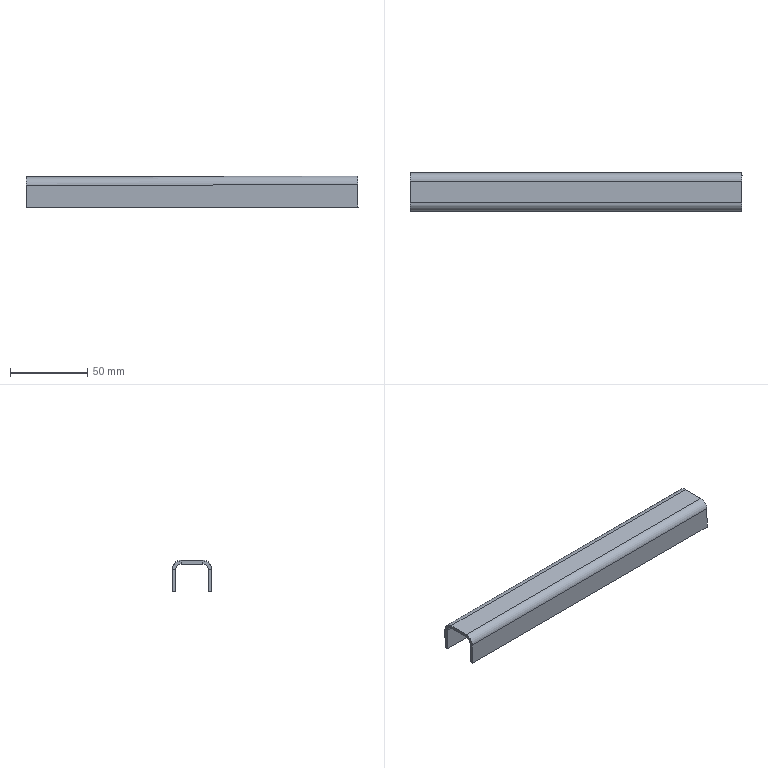Component | SolidWorks | LeftRearDoor-1_RearDoorUpperAndLowerReinforcementBar-1 | 1 solid | 22 faces | box 215.05 x 25 x 20.54 mm | volume 24569 mm3 | plane 18 | cylinder 4 | commonest cylinder face diameters 11 x2 7 x2 | material Malleable Cast Iron
STEP:
#1=COLOUR_RGB('',0.7922,0.8196,0.9333);
#2=FILL_AREA_STYLE_COLOUR('',#1);
#3=FILL_AREA_STYLE('',(#2));
#4=SURFACE_STYLE_FILL_AREA(#3);
#5=SURFACE_SIDE_STYLE('',(#4));
#6=SURFACE_STYLE_USAGE(.BOTH.,#5);
#7=PRESENTATION_STYLE_ASSIGNMENT((#6));
#8=CARTESIAN_POINT('',(9.361,73.502,-6.524));
#9=VERTEX_POINT('',#8);
#10=CARTESIAN_POINT('',(9.361,73.502,-6.603));
#11=VERTEX_POINT('',#10);
#12=CARTESIAN_POINT('',(9.361,73.502,-6.524));
#13=DIRECTION('',(0.002502,0.,-1.));
#14=VECTOR('',#13,39.37);
#15=LINE('',#12,#14);
#16=EDGE_CURVE('',#9,#11,#15,.T.);
#17=ORIENTED_EDGE('',*,*,#16,.F.);
#18=CARTESIAN_POINT('',(9.362,73.286,-6.741));
#19=VERTEX_POINT('',#18);
#20=CARTESIAN_POINT('',(9.362,73.502,-6.741));
#21=DIRECTION('',(-1.,-0.,-0.002502));
#22=DIRECTION('',(0.002502,0.,-1.));
#23=AXIS2_PLACEMENT_3D('',#20,#21,#22);
#24=CIRCLE('',#23,0.2165);
#25=EDGE_CURVE('',#19,#9,#24,.T.);
#26=ORIENTED_EDGE('',*,*,#25,.F.);
#27=CARTESIAN_POINT('',(9.362,73.365,-6.741));
#28=VERTEX_POINT('',#27);
#29=CARTESIAN_POINT('',(9.362,73.365,-6.741));
#30=DIRECTION('',(0.,-1.,-0.));
#31=VECTOR('',#30,39.37);
#32=LINE('',#29,#31);
#33=EDGE_CURVE('',#28,#19,#32,.T.);
#34=ORIENTED_EDGE('',*,*,#33,.F.);
#35=CARTESIAN_POINT('',(9.362,73.502,-6.741));
#36=DIRECTION('',(-1.,-0.,-0.002502));
#37=DIRECTION('',(0.,1.,0.));
#38=AXIS2_PLACEMENT_3D('',#35,#36,#37);
#39=CIRCLE('',#38,0.1378);
#40=EDGE_CURVE('',#28,#11,#39,.T.);
#41=ORIENTED_EDGE('',*,*,#40,.T.);
#42=EDGE_LOOP('',(#17,#26,#34,#41));
#43=FACE_OUTER_BOUND('',#42,.T.);
#44=CARTESIAN_POINT('',(9.361,73.502,-6.524));
#45=DIRECTION('',(1.,0.,0.002502));
#46=DIRECTION('',(0.002502,0.,-1.));
#47=AXIS2_PLACEMENT_3D('',#44,#45,#46);
#48=PLANE('',#47);
#49=ADVANCED_FACE('',(#43),#48,.T.);
#50=CARTESIAN_POINT('',(9.361,74.054,-6.524));
#51=VERTEX_POINT('',#50);
#52=CARTESIAN_POINT('',(9.361,73.286,-6.524));
#53=DIRECTION('',(-0.,1.,0.));
#54=VECTOR('',#53,39.37);
#55=LINE('',#52,#54);
#56=EDGE_CURVE('',#9,#51,#55,.T.);
#57=ORIENTED_EDGE('',*,*,#56,.F.);
#58=ORIENTED_EDGE('',*,*,#16,.T.);
#59=CARTESIAN_POINT('',(9.361,74.054,-6.603));
#60=VERTEX_POINT('',#59);
#61=CARTESIAN_POINT('',(9.361,73.286,-6.603));
#62=DIRECTION('',(-0.,1.,0.));
#63=VECTOR('',#62,39.37);
#64=LINE('',#61,#63);
#65=EDGE_CURVE('',#11,#60,#64,.T.);
#66=ORIENTED_EDGE('',*,*,#65,.T.);
#67=CARTESIAN_POINT('',(9.361,74.054,-6.603));
#68=DIRECTION('',(-0.002502,-0.,1.));
#69=VECTOR('',#68,39.37);
#70=LINE('',#67,#69);
#71=EDGE_CURVE('',#60,#51,#70,.T.);
#72=ORIENTED_EDGE('',*,*,#71,.T.);
#73=EDGE_LOOP('',(#57,#58,#66,#72));
#74=FACE_OUTER_BOUND('',#73,.T.);
#75=CARTESIAN_POINT('',(9.362,73.365,-6.741));
#76=DIRECTION('',(1.,0.,0.002502));
#77=DIRECTION('',(0.002502,0.,-1.));
#78=AXIS2_PLACEMENT_3D('',#75,#76,#77);
#79=PLANE('',#78);
#80=ADVANCED_FACE('',(#74),#79,.T.);
#81=CARTESIAN_POINT('',(0.897,73.286,-6.762));
#82=VERTEX_POINT('',#81);
#83=CARTESIAN_POINT('',(0.897,73.365,-6.762));
#84=VERTEX_POINT('',#83);
#85=CARTESIAN_POINT('',(0.897,73.286,-6.762));
#86=DIRECTION('',(-0.,1.,0.));
#87=VECTOR('',#86,39.37);
#88=LINE('',#85,#87);
#89=EDGE_CURVE('',#82,#84,#88,.T.);
#90=ORIENTED_EDGE('',*,*,#89,.F.);
#91=CARTESIAN_POINT('',(0.8965,73.502,-6.545));
#92=VERTEX_POINT('',#91);
#93=CARTESIAN_POINT('',(0.897,73.502,-6.762));
#94=DIRECTION('',(-1.,-0.,-0.002502));
#95=DIRECTION('',(0.002502,0.,-1.));
#96=AXIS2_PLACEMENT_3D('',#93,#94,#95);
#97=CIRCLE('',#96,0.2165);
#98=EDGE_CURVE('',#82,#92,#97,.T.);
#99=ORIENTED_EDGE('',*,*,#98,.T.);
#100=CARTESIAN_POINT('',(0.8967,73.502,-6.624));
#101=VERTEX_POINT('',#100);
#102=CARTESIAN_POINT('',(0.8967,73.502,-6.624));
#103=DIRECTION('',(-0.002502,-0.,1.));
#104=VECTOR('',#103,39.37);
#105=LINE('',#102,#104);
#106=EDGE_CURVE('',#101,#92,#105,.T.);
#107=ORIENTED_EDGE('',*,*,#106,.F.);
#108=CARTESIAN_POINT('',(0.897,73.502,-6.762));
#109=DIRECTION('',(-1.,-0.,-0.002502));
#110=DIRECTION('',(-0.,1.,0.));
#111=AXIS2_PLACEMENT_3D('',#108,#109,#110);
#112=CIRCLE('',#111,0.1378);
#113=EDGE_CURVE('',#84,#101,#112,.T.);
#114=ORIENTED_EDGE('',*,*,#113,.F.);
#115=EDGE_LOOP('',(#90,#99,#107,#114));
#116=FACE_OUTER_BOUND('',#115,.T.);
#117=CARTESIAN_POINT('',(0.897,73.286,-6.762));
#118=DIRECTION('',(-1.,-0.,-0.002502));
#119=DIRECTION('',(-0.002502,-0.,1.));
#120=AXIS2_PLACEMENT_3D('',#117,#118,#119);
#121=PLANE('',#120);
#122=ADVANCED_FACE('',(#116),#121,.T.);
#123=CARTESIAN_POINT('',(0.8984,73.286,-7.333));
#124=VERTEX_POINT('',#123);
#125=CARTESIAN_POINT('',(0.8984,73.286,-7.333));
#126=DIRECTION('',(-0.002502,-0.,1.));
#127=VECTOR('',#126,39.37);
#128=LINE('',#125,#127);
#129=EDGE_CURVE('',#124,#82,#128,.T.);
#130=ORIENTED_EDGE('',*,*,#129,.T.);
#131=ORIENTED_EDGE('',*,*,#89,.T.);
#132=CARTESIAN_POINT('',(0.8984,73.365,-7.333));
#133=VERTEX_POINT('',#132);
#134=CARTESIAN_POINT('',(0.8984,73.365,-7.333));
#135=DIRECTION('',(-0.002502,-0.,1.));
#136=VECTOR('',#135,39.37);
#137=LINE('',#134,#136);
#138=EDGE_CURVE('',#133,#84,#137,.T.);
#139=ORIENTED_EDGE('',*,*,#138,.F.);
#140=CARTESIAN_POINT('',(0.8984,73.365,-7.333));
#141=DIRECTION('',(0.,-1.,-0.));
#142=VECTOR('',#141,39.37);
#143=LINE('',#140,#142);
#144=EDGE_CURVE('',#133,#124,#143,.T.);
#145=ORIENTED_EDGE('',*,*,#144,.T.);
#146=EDGE_LOOP('',(#130,#131,#139,#145));
#147=FACE_OUTER_BOUND('',#146,.T.);
#148=CARTESIAN_POINT('',(0.8967,73.502,-6.624));
#149=DIRECTION('',(-1.,-0.,-0.002502));
#150=DIRECTION('',(-0.002502,-0.,1.));
#151=AXIS2_PLACEMENT_3D('',#148,#149,#150);
#152=PLANE('',#151);
#153=ADVANCED_FACE('',(#147),#152,.T.);
#154=CARTESIAN_POINT('',(9.362,74.27,-6.741));
#155=VERTEX_POINT('',#154);
#156=CARTESIAN_POINT('',(9.362,74.191,-6.741));
#157=VERTEX_POINT('',#156);
#158=CARTESIAN_POINT('',(9.362,74.27,-6.741));
#159=DIRECTION('',(0.,-1.,-0.));
#160=VECTOR('',#159,39.37);
#161=LINE('',#158,#160);
#162=EDGE_CURVE('',#155,#157,#161,.T.);
#163=ORIENTED_EDGE('',*,*,#162,.F.);
#164=CARTESIAN_POINT('',(9.362,74.054,-6.741));
#165=DIRECTION('',(-1.,-0.,-0.002502));
#166=DIRECTION('',(0.002502,0.,-1.));
#167=AXIS2_PLACEMENT_3D('',#164,#165,#166);
#168=CIRCLE('',#167,0.2165);
#169=EDGE_CURVE('',#51,#155,#168,.T.);
#170=ORIENTED_EDGE('',*,*,#169,.F.);
#171=ORIENTED_EDGE('',*,*,#71,.F.);
#172=CARTESIAN_POINT('',(9.362,74.054,-6.741));
#173=DIRECTION('',(-1.,-0.,-0.002502));
#174=DIRECTION('',(0.,1.,0.));
#175=AXIS2_PLACEMENT_3D('',#172,#173,#174);
#176=CIRCLE('',#175,0.1378);
#177=EDGE_CURVE('',#60,#157,#176,.T.);
#178=ORIENTED_EDGE('',*,*,#177,.T.);
#179=EDGE_LOOP('',(#163,#170,#171,#178));
#180=FACE_OUTER_BOUND('',#179,.T.);
#181=CARTESIAN_POINT('',(9.362,74.27,-6.741));
#182=DIRECTION('',(1.,0.,0.002502));
#183=DIRECTION('',(0.002502,0.,-1.));
#184=AXIS2_PLACEMENT_3D('',#181,#182,#183);
#185=PLANE('',#184);
#186=ADVANCED_FACE('',(#180),#185,.T.);
#187=CARTESIAN_POINT('',(9.363,74.27,-7.312));
#188=VERTEX_POINT('',#187);
#189=CARTESIAN_POINT('',(9.361,74.27,-6.524));
#190=DIRECTION('',(0.002502,0.,-1.));
#191=VECTOR('',#190,39.37);
#192=LINE('',#189,#191);
#193=EDGE_CURVE('',#155,#188,#192,.T.);
#194=ORIENTED_EDGE('',*,*,#193,.F.);
#195=ORIENTED_EDGE('',*,*,#162,.T.);
#196=CARTESIAN_POINT('',(9.363,74.191,-7.312));
#197=VERTEX_POINT('',#196);
#198=CARTESIAN_POINT('',(9.361,74.191,-6.524));
#199=DIRECTION('',(0.002502,0.,-1.));
#200=VECTOR('',#199,39.37);
#201=LINE('',#198,#200);
#202=EDGE_CURVE('',#157,#197,#201,.T.);
#203=ORIENTED_EDGE('',*,*,#202,.T.);
#204=CARTESIAN_POINT('',(9.363,74.27,-7.312));
#205=DIRECTION('',(0.,-1.,-0.));
#206=VECTOR('',#205,39.37);
#207=LINE('',#204,#206);
#208=EDGE_CURVE('',#188,#197,#207,.T.);
#209=ORIENTED_EDGE('',*,*,#208,.F.);
#210=EDGE_LOOP('',(#194,#195,#203,#209));
#211=FACE_OUTER_BOUND('',#210,.T.);
#212=CARTESIAN_POINT('',(9.361,74.054,-6.603));
#213=DIRECTION('',(1.,0.,0.002502));
#214=DIRECTION('',(0.002502,0.,-1.));
#215=AXIS2_PLACEMENT_3D('',#212,#213,#214);
#216=PLANE('',#215);
#217=ADVANCED_FACE('',(#211),#216,.T.);
#218=CARTESIAN_POINT('',(0.8965,74.054,-6.545));
#219=VERTEX_POINT('',#218);
#220=CARTESIAN_POINT('',(0.8967,74.054,-6.624));
#221=VERTEX_POINT('',#220);
#222=CARTESIAN_POINT('',(0.8965,74.054,-6.545));
#223=DIRECTION('',(0.002502,0.,-1.));
#224=VECTOR('',#223,39.37);
#225=LINE('',#222,#224);
#226=EDGE_CURVE('',#219,#221,#225,.T.);
#227=ORIENTED_EDGE('',*,*,#226,.F.);
#228=CARTESIAN_POINT('',(0.897,74.27,-6.762));
#229=VERTEX_POINT('',#228);
#230=CARTESIAN_POINT('',(0.897,74.054,-6.762));
#231=DIRECTION('',(-1.,-0.,-0.002502));
#232=DIRECTION('',(0.002502,0.,-1.));
#233=AXIS2_PLACEMENT_3D('',#230,#231,#232);
#234=CIRCLE('',#233,0.2165);
#235=EDGE_CURVE('',#219,#229,#234,.T.);
#236=ORIENTED_EDGE('',*,*,#235,.T.);
#237=CARTESIAN_POINT('',(0.897,74.191,-6.762));
#238=VERTEX_POINT('',#237);
#239=CARTESIAN_POINT('',(0.897,74.191,-6.762));
#240=DIRECTION('',(-0.,1.,0.));
#241=VECTOR('',#240,39.37);
#242=LINE('',#239,#241);
#243=EDGE_CURVE('',#238,#229,#242,.T.);
#244=ORIENTED_EDGE('',*,*,#243,.F.);
#245=CARTESIAN_POINT('',(0.897,74.054,-6.762));
#246=DIRECTION('',(-1.,-0.,-0.002502));
#247=DIRECTION('',(-0.,1.,0.));
#248=AXIS2_PLACEMENT_3D('',#245,#246,#247);
#249=CIRCLE('',#248,0.1378);
#250=EDGE_CURVE('',#221,#238,#249,.T.);
#251=ORIENTED_EDGE('',*,*,#250,.F.);
#252=EDGE_LOOP('',(#227,#236,#244,#251));
#253=FACE_OUTER_BOUND('',#252,.T.);
#254=CARTESIAN_POINT('',(0.8965,74.054,-6.545));
#255=DIRECTION('',(-1.,-0.,-0.002502));
#256=DIRECTION('',(-0.002502,-0.,1.));
#257=AXIS2_PLACEMENT_3D('',#254,#255,#256);
#258=PLANE('',#257);
#259=ADVANCED_FACE('',(#253),#258,.T.);
#260=CARTESIAN_POINT('',(0.8965,73.286,-6.545));
#261=DIRECTION('',(-0.,1.,0.));
#262=VECTOR('',#261,39.37);
#263=LINE('',#260,#262);
#264=EDGE_CURVE('',#92,#219,#263,.T.);
#265=ORIENTED_EDGE('',*,*,#264,.T.);
#266=ORIENTED_EDGE('',*,*,#226,.T.);
#267=CARTESIAN_POINT('',(0.8967,73.286,-6.624));
#268=DIRECTION('',(-0.,1.,0.));
#269=VECTOR('',#268,39.37);
#270=LINE('',#267,#269);
#271=EDGE_CURVE('',#101,#221,#270,.T.);
#272=ORIENTED_EDGE('',*,*,#271,.F.);
#273=ORIENTED_EDGE('',*,*,#106,.T.);
#274=EDGE_LOOP('',(#265,#266,#272,#273));
#275=FACE_OUTER_BOUND('',#274,.T.);
#276=CARTESIAN_POINT('',(0.897,74.191,-6.762));
#277=DIRECTION('',(-1.,-0.,-0.002502));
#278=DIRECTION('',(-0.002502,-0.,1.));
#279=AXIS2_PLACEMENT_3D('',#276,#277,#278);
#280=PLANE('',#279);
#281=ADVANCED_FACE('',(#275),#280,.T.);
#282=CARTESIAN_POINT('',(0.8984,74.191,-7.333));
#283=VERTEX_POINT('',#282);
#284=CARTESIAN_POINT('',(0.8965,74.191,-6.545));
#285=DIRECTION('',(0.002502,0.,-1.));
#286=VECTOR('',#285,39.37);
#287=LINE('',#284,#286);
#288=EDGE_CURVE('',#238,#283,#287,.T.);
#289=ORIENTED_EDGE('',*,*,#288,.T.);
#290=CARTESIAN_POINT('',(9.363,74.191,-7.312));
#291=DIRECTION('',(-1.,-0.,-0.002502));
#292=VECTOR('',#291,39.37);
#293=LINE('',#290,#292);
#294=EDGE_CURVE('',#197,#283,#293,.T.);
#295=ORIENTED_EDGE('',*,*,#294,.F.);
#296=ORIENTED_EDGE('',*,*,#202,.F.);
#297=CARTESIAN_POINT('',(9.362,74.191,-6.741));
#298=DIRECTION('',(-1.,-0.,-0.002502));
#299=VECTOR('',#298,39.37);
#300=LINE('',#297,#299);
#301=EDGE_CURVE('',#157,#238,#300,.T.);
#302=ORIENTED_EDGE('',*,*,#301,.T.);
#303=EDGE_LOOP('',(#289,#295,#296,#302));
#304=FACE_OUTER_BOUND('',#303,.T.);
#305=CARTESIAN_POINT('',(9.361,74.191,-6.524));
#306=DIRECTION('',(-0.,1.,0.));
#307=DIRECTION('',(-0.002502,-0.,1.));
#308=AXIS2_PLACEMENT_3D('',#305,#306,#307);
#309=PLANE('',#308);
#310=ADVANCED_FACE('',(#304),#309,.F.);
#311=CARTESIAN_POINT('',(0.8984,74.27,-7.333));
#312=VERTEX_POINT('',#311);
#313=CARTESIAN_POINT('',(0.8984,74.27,-7.333));
#314=DIRECTION('',(0.,-1.,-0.));
#315=VECTOR('',#314,39.37);
#316=LINE('',#313,#315);
#317=EDGE_CURVE('',#312,#283,#316,.T.);
#318=ORIENTED_EDGE('',*,*,#317,.F.);
#319=CARTESIAN_POINT('',(9.363,74.27,-7.312));
#320=DIRECTION('',(-1.,-0.,-0.002502));
#321=VECTOR('',#320,39.37);
#322=LINE('',#319,#321);
#323=EDGE_CURVE('',#188,#312,#322,.T.);
#324=ORIENTED_EDGE('',*,*,#323,.F.);
#325=ORIENTED_EDGE('',*,*,#208,.T.);
#326=ORIENTED_EDGE('',*,*,#294,.T.);
#327=EDGE_LOOP('',(#318,#324,#325,#326));
#328=FACE_OUTER_BOUND('',#327,.T.);
#329=CARTESIAN_POINT('',(9.363,74.27,-7.312));
#330=DIRECTION('',(0.002502,0.,-1.));
#331=DIRECTION('',(-0.,1.,0.));
#332=AXIS2_PLACEMENT_3D('',#329,#330,#331);
#333=PLANE('',#332);
#334=ADVANCED_FACE('',(#328),#333,.T.);
#335=CARTESIAN_POINT('',(0.8965,74.27,-6.545));
#336=DIRECTION('',(0.002502,0.,-1.));
#337=VECTOR('',#336,39.37);
#338=LINE('',#335,#337);
#339=EDGE_CURVE('',#229,#312,#338,.T.);
#340=ORIENTED_EDGE('',*,*,#339,.F.);
#341=CARTESIAN_POINT('',(9.362,74.27,-6.741));
#342=DIRECTION('',(-1.,-0.,-0.002502));
#343=VECTOR('',#342,39.37);
#344=LINE('',#341,#343);
#345=EDGE_CURVE('',#155,#229,#344,.T.);
#346=ORIENTED_EDGE('',*,*,#345,.F.);
#347=ORIENTED_EDGE('',*,*,#193,.T.);
#348=ORIENTED_EDGE('',*,*,#323,.T.);
#349=EDGE_LOOP('',(#340,#346,#347,#348));
#350=FACE_OUTER_BOUND('',#349,.T.);
#351=CARTESIAN_POINT('',(9.361,74.27,-6.524));
#352=DIRECTION('',(-0.,1.,0.));
#353=DIRECTION('',(-0.002502,-0.,1.));
#354=AXIS2_PLACEMENT_3D('',#351,#352,#353);
#355=PLANE('',#354);
#356=ADVANCED_FACE('',(#350),#355,.T.);
#357=ORIENTED_EDGE('',*,*,#235,.F.);
#358=CARTESIAN_POINT('',(9.361,74.054,-6.524));
#359=DIRECTION('',(-1.,-0.,-0.002502));
#360=VECTOR('',#359,39.37);
#361=LINE('',#358,#360);
#362=EDGE_CURVE('',#51,#219,#361,.T.);
#363=ORIENTED_EDGE('',*,*,#362,.F.);
#364=ORIENTED_EDGE('',*,*,#169,.T.);
#365=ORIENTED_EDGE('',*,*,#345,.T.);
#366=EDGE_LOOP('',(#357,#363,#364,#365));
#367=FACE_OUTER_BOUND('',#366,.T.);
#368=CARTESIAN_POINT('',(9.362,74.054,-6.741));
#369=DIRECTION('',(-1.,-0.,-0.002502));
#370=DIRECTION('',(-0.002502,0.,1.));
#371=AXIS2_PLACEMENT_3D('',#368,#369,#370);
#372=CYLINDRICAL_SURFACE('',#371,0.2165);
#373=ADVANCED_FACE('',(#367),#372,.T.);
#374=ORIENTED_EDGE('',*,*,#264,.F.);
#375=CARTESIAN_POINT('',(9.361,73.502,-6.524));
#376=DIRECTION('',(-1.,-0.,-0.002502));
#377=VECTOR('',#376,39.37);
#378=LINE('',#375,#377);
#379=EDGE_CURVE('',#9,#92,#378,.T.);
#380=ORIENTED_EDGE('',*,*,#379,.F.);
#381=ORIENTED_EDGE('',*,*,#56,.T.);
#382=ORIENTED_EDGE('',*,*,#362,.T.);
#383=EDGE_LOOP('',(#374,#380,#381,#382));
#384=FACE_OUTER_BOUND('',#383,.T.);
#385=CARTESIAN_POINT('',(9.361,73.286,-6.524));
#386=DIRECTION('',(-0.002502,-0.,1.));
#387=DIRECTION('',(0.,-1.,-0.));
#388=AXIS2_PLACEMENT_3D('',#385,#386,#387);
#389=PLANE('',#388);
#390=ADVANCED_FACE('',(#384),#389,.T.);
#391=ORIENTED_EDGE('',*,*,#98,.F.);
#392=CARTESIAN_POINT('',(9.362,73.286,-6.741));
#393=DIRECTION('',(-1.,-0.,-0.002502));
#394=VECTOR('',#393,39.37);
#395=LINE('',#392,#394);
#396=EDGE_CURVE('',#19,#82,#395,.T.);
#397=ORIENTED_EDGE('',*,*,#396,.F.);
#398=ORIENTED_EDGE('',*,*,#25,.T.);
#399=ORIENTED_EDGE('',*,*,#379,.T.);
#400=EDGE_LOOP('',(#391,#397,#398,#399));
#401=FACE_OUTER_BOUND('',#400,.T.);
#402=CARTESIAN_POINT('',(9.362,73.502,-6.741));
#403=DIRECTION('',(-1.,-0.,-0.002502));
#404=DIRECTION('',(-0.002502,0.,1.));
#405=AXIS2_PLACEMENT_3D('',#402,#403,#404);
#406=CYLINDRICAL_SURFACE('',#405,0.2165);
#407=ADVANCED_FACE('',(#401),#406,.T.);
#408=ORIENTED_EDGE('',*,*,#129,.F.);
#409=CARTESIAN_POINT('',(9.363,73.286,-7.312));
#410=VERTEX_POINT('',#409);
#411=CARTESIAN_POINT('',(9.363,73.286,-7.312));
#412=DIRECTION('',(-1.,-0.,-0.002502));
#413=VECTOR('',#412,39.37);
#414=LINE('',#411,#413);
#415=EDGE_CURVE('',#410,#124,#414,.T.);
#416=ORIENTED_EDGE('',*,*,#415,.F.);
#417=CARTESIAN_POINT('',(9.363,73.286,-7.312));
#418=DIRECTION('',(-0.002502,-0.,1.));
#419=VECTOR('',#418,39.37);
#420=LINE('',#417,#419);
#421=EDGE_CURVE('',#410,#19,#420,.T.);
#422=ORIENTED_EDGE('',*,*,#421,.T.);
#423=ORIENTED_EDGE('',*,*,#396,.T.);
#424=EDGE_LOOP('',(#408,#416,#422,#423));
#425=FACE_OUTER_BOUND('',#424,.T.);
#426=CARTESIAN_POINT('',(9.363,73.286,-7.312));
#427=DIRECTION('',(0.,-1.,-0.));
#428=DIRECTION('',(0.002502,0.,-1.));
#429=AXIS2_PLACEMENT_3D('',#426,#427,#428);
#430=PLANE('',#429);
#431=ADVANCED_FACE('',(#425),#430,.T.);
#432=ORIENTED_EDGE('',*,*,#144,.F.);
#433=CARTESIAN_POINT('',(9.363,73.365,-7.312));
#434=VERTEX_POINT('',#433);
#435=CARTESIAN_POINT('',(9.363,73.365,-7.312));
#436=DIRECTION('',(-1.,-0.,-0.002502));
#437=VECTOR('',#436,39.37);
#438=LINE('',#435,#437);
#439=EDGE_CURVE('',#434,#133,#438,.T.);
#440=ORIENTED_EDGE('',*,*,#439,.F.);
#441=CARTESIAN_POINT('',(9.363,73.365,-7.312));
#442=DIRECTION('',(0.,-1.,-0.));
#443=VECTOR('',#442,39.37);
#444=LINE('',#441,#443);
#445=EDGE_CURVE('',#434,#410,#444,.T.);
#446=ORIENTED_EDGE('',*,*,#445,.T.);
#447=ORIENTED_EDGE('',*,*,#415,.T.);
#448=EDGE_LOOP('',(#432,#440,#446,#447));
#449=FACE_OUTER_BOUND('',#448,.T.);
#450=CARTESIAN_POINT('',(9.363,73.365,-7.312));
#451=DIRECTION('',(0.002502,0.,-1.));
#452=DIRECTION('',(-0.,1.,0.));
#453=AXIS2_PLACEMENT_3D('',#450,#451,#452);
#454=PLANE('',#453);
#455=ADVANCED_FACE('',(#449),#454,.T.);
#456=ORIENTED_EDGE('',*,*,#138,.T.);
#457=CARTESIAN_POINT('',(9.362,73.365,-6.741));
#458=DIRECTION('',(-1.,-0.,-0.002502));
#459=VECTOR('',#458,39.37);
#460=LINE('',#457,#459);
#461=EDGE_CURVE('',#28,#84,#460,.T.);
#462=ORIENTED_EDGE('',*,*,#461,.F.);
#463=CARTESIAN_POINT('',(9.363,73.365,-7.312));
#464=DIRECTION('',(-0.002502,-0.,1.));
#465=VECTOR('',#464,39.37);
#466=LINE('',#463,#465);
#467=EDGE_CURVE('',#434,#28,#466,.T.);
#468=ORIENTED_EDGE('',*,*,#467,.F.);
#469=ORIENTED_EDGE('',*,*,#439,.T.);
#470=EDGE_LOOP('',(#456,#462,#468,#469));
#471=FACE_OUTER_BOUND('',#470,.T.);
#472=CARTESIAN_POINT('',(9.363,73.365,-7.312));
#473=DIRECTION('',(0.,-1.,-0.));
#474=DIRECTION('',(0.002502,0.,-1.));
#475=AXIS2_PLACEMENT_3D('',#472,#473,#474);
#476=PLANE('',#475);
#477=ADVANCED_FACE('',(#471),#476,.F.);
#478=ORIENTED_EDGE('',*,*,#113,.T.);
#479=CARTESIAN_POINT('',(9.361,73.502,-6.603));
#480=DIRECTION('',(-1.,-0.,-0.002502));
#481=VECTOR('',#480,39.37);
#482=LINE('',#479,#481);
#483=EDGE_CURVE('',#11,#101,#482,.T.);
#484=ORIENTED_EDGE('',*,*,#483,.F.);
#485=ORIENTED_EDGE('',*,*,#40,.F.);
#486=ORIENTED_EDGE('',*,*,#461,.T.);
#487=EDGE_LOOP('',(#478,#484,#485,#486));
#488=FACE_OUTER_BOUND('',#487,.T.);
#489=CARTESIAN_POINT('',(9.362,73.502,-6.741));
#490=DIRECTION('',(-1.,-0.,-0.002502));
#491=DIRECTION('',(-0.002502,0.,1.));
#492=AXIS2_PLACEMENT_3D('',#489,#490,#491);
#493=CYLINDRICAL_SURFACE('',#492,0.1378);
#494=ADVANCED_FACE('',(#488),#493,.F.);
#495=ORIENTED_EDGE('',*,*,#271,.T.);
#496=CARTESIAN_POINT('',(9.361,74.054,-6.603));
#497=DIRECTION('',(-1.,-0.,-0.002502));
#498=VECTOR('',#497,39.37);
#499=LINE('',#496,#498);
#500=EDGE_CURVE('',#60,#221,#499,.T.);
#501=ORIENTED_EDGE('',*,*,#500,.F.);
#502=ORIENTED_EDGE('',*,*,#65,.F.);
#503=ORIENTED_EDGE('',*,*,#483,.T.);
#504=EDGE_LOOP('',(#495,#501,#502,#503));
#505=FACE_OUTER_BOUND('',#504,.T.);
#506=CARTESIAN_POINT('',(9.361,73.286,-6.603));
#507=DIRECTION('',(-0.002502,-0.,1.));
#508=DIRECTION('',(0.,-1.,-0.));
#509=AXIS2_PLACEMENT_3D('',#506,#507,#508);
#510=PLANE('',#509);
#511=ADVANCED_FACE('',(#505),#510,.F.);
#512=ORIENTED_EDGE('',*,*,#250,.T.);
#513=ORIENTED_EDGE('',*,*,#301,.F.);
#514=ORIENTED_EDGE('',*,*,#177,.F.);
#515=ORIENTED_EDGE('',*,*,#500,.T.);
#516=EDGE_LOOP('',(#512,#513,#514,#515));
#517=FACE_OUTER_BOUND('',#516,.T.);
#518=CARTESIAN_POINT('',(9.362,74.054,-6.741));
#519=DIRECTION('',(-1.,-0.,-0.002502));
#520=DIRECTION('',(-0.002502,0.,1.));
#521=AXIS2_PLACEMENT_3D('',#518,#519,#520);
#522=CYLINDRICAL_SURFACE('',#521,0.1378);
#523=ADVANCED_FACE('',(#517),#522,.F.);
#524=ORIENTED_EDGE('',*,*,#467,.T.);
#525=ORIENTED_EDGE('',*,*,#33,.T.);
#526=ORIENTED_EDGE('',*,*,#421,.F.);
#527=ORIENTED_EDGE('',*,*,#445,.F.);
#528=EDGE_LOOP('',(#524,#525,#526,#527));
#529=FACE_OUTER_BOUND('',#528,.T.);
#530=CARTESIAN_POINT('',(9.362,74.054,-6.741));
#531=DIRECTION('',(1.,0.,0.002502));
#532=DIRECTION('',(-0.,1.,0.));
#533=AXIS2_PLACEMENT_3D('',#530,#531,#532);
#534=PLANE('',#533);
#535=ADVANCED_FACE('',(#529),#534,.T.);
#536=ORIENTED_EDGE('',*,*,#288,.F.);
#537=ORIENTED_EDGE('',*,*,#243,.T.);
#538=ORIENTED_EDGE('',*,*,#339,.T.);
#539=ORIENTED_EDGE('',*,*,#317,.T.);
#540=EDGE_LOOP('',(#536,#537,#538,#539));
#541=FACE_OUTER_BOUND('',#540,.T.);
#542=CARTESIAN_POINT('',(0.897,74.054,-6.762));
#543=DIRECTION('',(1.,0.,0.002502));
#544=DIRECTION('',(-0.,1.,0.));
#545=AXIS2_PLACEMENT_3D('',#542,#543,#544);
#546=PLANE('',#545);
#547=ADVANCED_FACE('',(#541),#546,.F.);
#548=CLOSED_SHELL('',(#49,#80,#122,#153,#186,#217,#259,#281,#310,#334,#356,#373,#390,#407,#431,#455,#477,#494,#511,#523,#535,#547));
#549=MANIFOLD_SOLID_BREP('',#548);
#550=STYLED_ITEM('',(#7),#549);
#551=(LENGTH_UNIT()NAMED_UNIT(*)SI_UNIT($,.METRE.));
#552=LENGTH_MEASURE_WITH_UNIT(LENGTH_MEASURE(0.0254),#551);
#553=DIMENSIONAL_EXPONENTS(1.,0.,0.,0.,0.,0.,0.);
#554=(CONVERSION_BASED_UNIT('',#552)LENGTH_UNIT()NAMED_UNIT(#553));
#555=UNCERTAINTY_MEASURE_WITH_UNIT(LENGTH_MEASURE(0.00001),#554,'','');
#556=(NAMED_UNIT(*)PLANE_ANGLE_UNIT()SI_UNIT($,.RADIAN.));
#557=(NAMED_UNIT(*)SI_UNIT($,.STERADIAN.)SOLID_ANGLE_UNIT());
#558=(GEOMETRIC_REPRESENTATION_CONTEXT(3)GLOBAL_UNCERTAINTY_ASSIGNED_CONTEXT((#555))GLOBAL_UNIT_ASSIGNED_CONTEXT((#554,#556,#557))REPRESENTATION_CONTEXT('',''));
#559=MECHANICAL_DESIGN_GEOMETRIC_PRESENTATION_REPRESENTATION('',(#550),#558);
#560=CARTESIAN_POINT('',(0.,0.,0.));
#561=DIRECTION('',(0.,0.,1.));
#562=DIRECTION('',(1.,0.,0.));
#563=AXIS2_PLACEMENT_3D('',#560,#561,#562);
#564=(LENGTH_UNIT()NAMED_UNIT(*)SI_UNIT($,.METRE.));
#565=LENGTH_MEASURE_WITH_UNIT(LENGTH_MEASURE(0.0254),#564);
#566=DIMENSIONAL_EXPONENTS(1.,0.,0.,0.,0.,0.,0.);
#567=(CONVERSION_BASED_UNIT('',#565)LENGTH_UNIT()NAMED_UNIT(#566));
#568=UNCERTAINTY_MEASURE_WITH_UNIT(LENGTH_MEASURE(0.00001),#567,'','');
#569=(NAMED_UNIT(*)PLANE_ANGLE_UNIT()SI_UNIT($,.RADIAN.));
#570=(NAMED_UNIT(*)SI_UNIT($,.STERADIAN.)SOLID_ANGLE_UNIT());
#571=(GEOMETRIC_REPRESENTATION_CONTEXT(3)GLOBAL_UNCERTAINTY_ASSIGNED_CONTEXT((#568))GLOBAL_UNIT_ASSIGNED_CONTEXT((#567,#569,#570))REPRESENTATION_CONTEXT('',''));
#572=ADVANCED_BREP_SHAPE_REPRESENTATION('',(#549,#563),#571);
#573=PRESENTATION_LAYER_ASSIGNMENT('','',(#550));